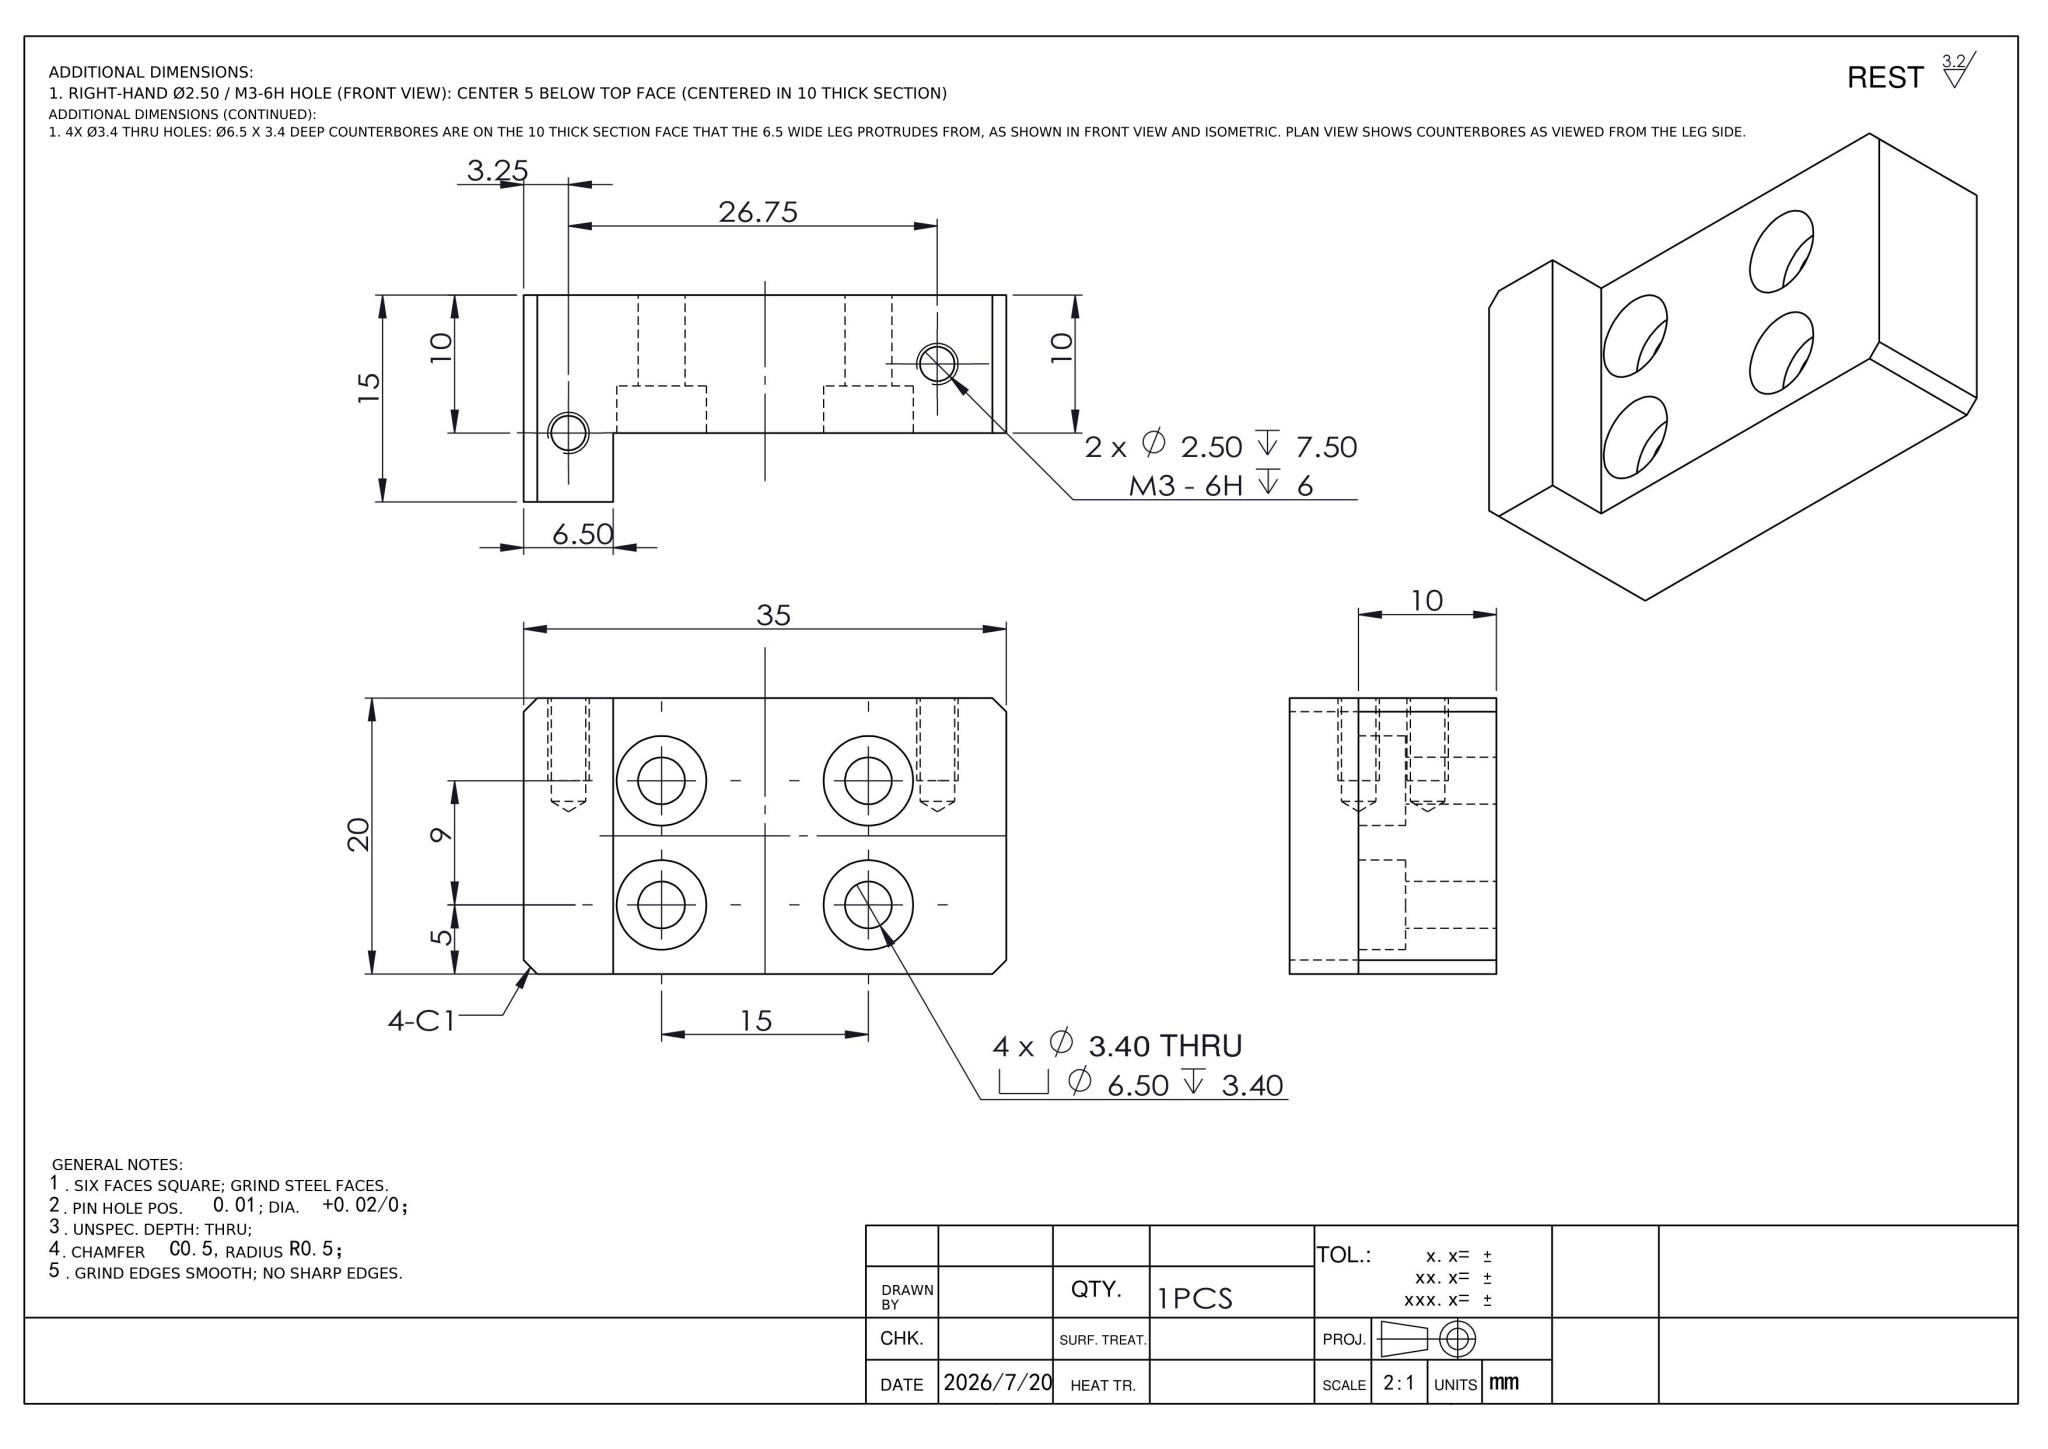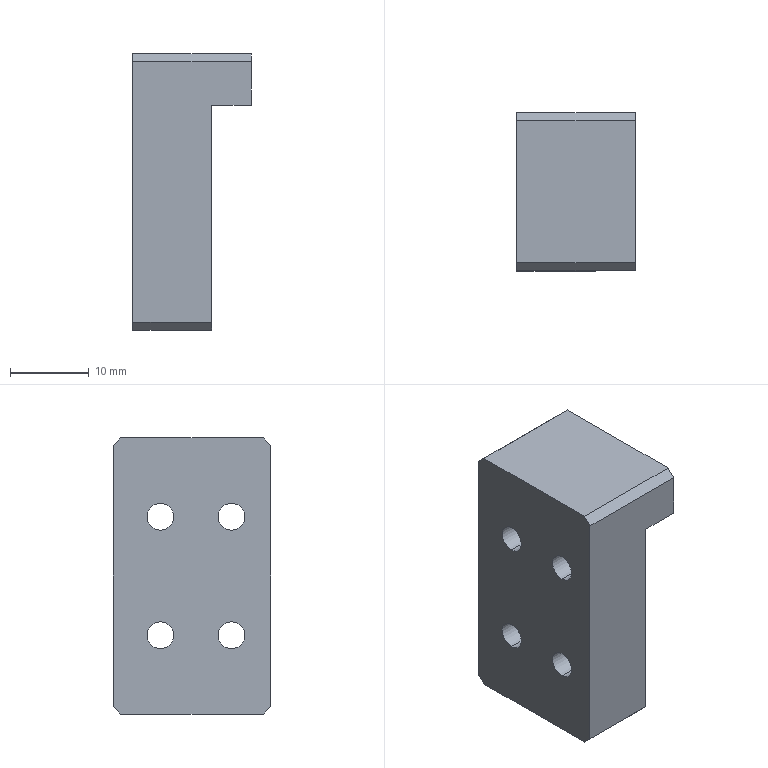Part | NX | mm | 1 solid | 40 faces | box 15 x 20 x 35 mm | volume 6858 mm3 | cylinder 20 | plane 16 | cone 4 | commonest cylinder face diameters 6.5 x8 3.4 x8 2.5 x4